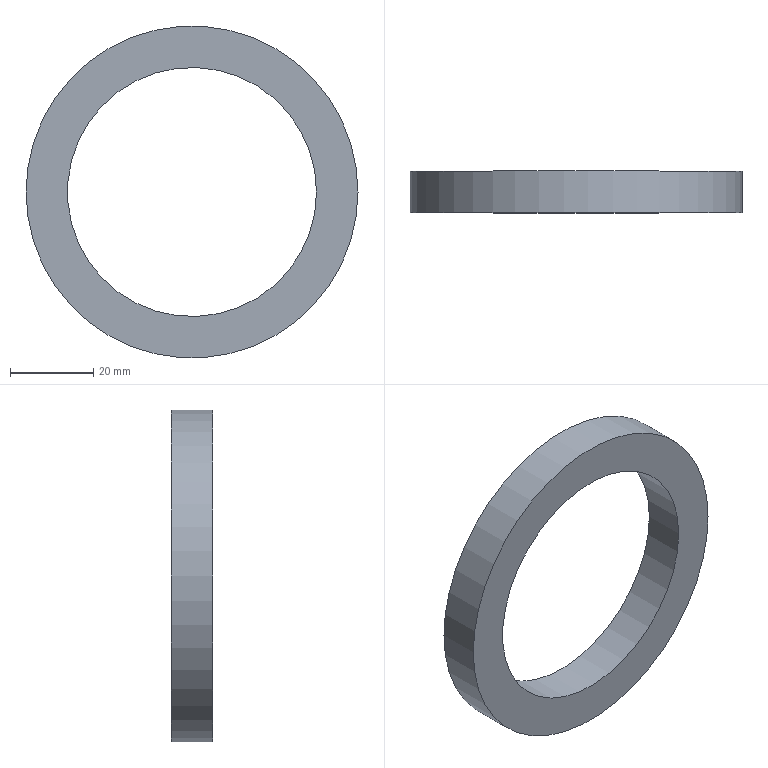Component | NX | OIL_SEAL_80X60X10 | 1 solid | 4 faces | box 80 x 10 x 80 mm | volume 21991 mm3 | cylinder 2 | plane 2 | commonest cylinder face diameters 80 x1 60 x1
STEP:
#1=CARTESIAN_POINT('',(0.,0.,0.));
#2=DIRECTION('',(0.,0.,1.));
#3=DIRECTION('',(1.,0.,0.));
#4=AXIS2_PLACEMENT_3D('',#1,#2,#3);
#5=CARTESIAN_POINT('',(45.,-94.6,-249.5));
#6=VERTEX_POINT('',#5);
#7=CARTESIAN_POINT('',(5.,-94.6,-249.5));
#8=DIRECTION('',(0.,-1.,0.));
#9=DIRECTION('',(1.,0.,0.));
#10=AXIS2_PLACEMENT_3D('',#7,#8,#9);
#11=CIRCLE('',#10,40.);
#12=CARTESIAN_POINT('',(5.,-94.6,-249.5));
#13=DIRECTION('',(0.,1.,0.));
#14=DIRECTION('',(-1.,0.,0.));
#15=AXIS2_PLACEMENT_3D('',#12,#13,#14);
#16=CYLINDRICAL_SURFACE('',#15,40.);
#17=CARTESIAN_POINT('',(9.425,0.));
#18=DIRECTION('',(-1.,0.));
#19=VECTOR('',#18,1.);
#20=LINE('',#17,#19);
#21=(GEOMETRIC_REPRESENTATION_CONTEXT(2)PARAMETRIC_REPRESENTATION_CONTEXT()REPRESENTATION_CONTEXT('',''));
#22=DEFINITIONAL_REPRESENTATION('',(#20),#21);
#23=PCURVE('',#16,#22);
#24=CARTESIAN_POINT('',(5.,-94.6,-249.5));
#25=DIRECTION('',(0.,-1.,0.));
#26=DIRECTION('',(1.,0.,0.));
#27=AXIS2_PLACEMENT_3D('',#24,#25,#26);
#28=PLANE('',#27);
#29=CARTESIAN_POINT('',(0.,0.));
#30=DIRECTION('',(1.,0.));
#31=AXIS2_PLACEMENT_2D('',#29,#30);
#32=CIRCLE('',#31,40.);
#33=(GEOMETRIC_REPRESENTATION_CONTEXT(2)PARAMETRIC_REPRESENTATION_CONTEXT()REPRESENTATION_CONTEXT('',''));
#34=DEFINITIONAL_REPRESENTATION('',(#32),#33);
#35=PCURVE('',#28,#34);
#36=SURFACE_CURVE('',#11,(#23,#35),.PCURVE_S1.);
#37=EDGE_CURVE('',#6,#6,#36,.T.);
#38=ORIENTED_EDGE('',*,*,#37,.F.);
#39=CARTESIAN_POINT('',(45.,-84.6,-249.5));
#40=VERTEX_POINT('',#39);
#41=CARTESIAN_POINT('',(45.,-94.6,-249.5));
#42=CARTESIAN_POINT('',(45.,-84.6,-249.5));
#43=B_SPLINE_CURVE_WITH_KNOTS('',1,(#41,#42),.UNSPECIFIED.,.F.,.F.,(2,2),(0.,10.),.PIECEWISE_BEZIER_KNOTS.);
#44=CARTESIAN_POINT('',(9.425,0.));
#45=DIRECTION('',(0.,1.));
#46=VECTOR('',#45,1.);
#47=LINE('',#44,#46);
#48=(GEOMETRIC_REPRESENTATION_CONTEXT(2)PARAMETRIC_REPRESENTATION_CONTEXT()REPRESENTATION_CONTEXT('',''));
#49=DEFINITIONAL_REPRESENTATION('',(#47),#48);
#50=PCURVE('',#16,#49);
#51=CARTESIAN_POINT('',(3.142,0.));
#52=DIRECTION('',(0.,1.));
#53=VECTOR('',#52,1.);
#54=LINE('',#51,#53);
#55=(GEOMETRIC_REPRESENTATION_CONTEXT(2)PARAMETRIC_REPRESENTATION_CONTEXT()REPRESENTATION_CONTEXT('',''));
#56=DEFINITIONAL_REPRESENTATION('',(#54),#55);
#57=PCURVE('',#16,#56);
#58=SEAM_CURVE('',#43,(#50,#57),.PCURVE_S1.);
#59=EDGE_CURVE('',#6,#40,#58,.T.);
#60=ORIENTED_EDGE('',*,*,#59,.T.);
#61=CARTESIAN_POINT('',(5.,-84.6,-249.5));
#62=DIRECTION('',(0.,-1.,0.));
#63=DIRECTION('',(1.,0.,0.));
#64=AXIS2_PLACEMENT_3D('',#61,#62,#63);
#65=CIRCLE('',#64,40.);
#66=CARTESIAN_POINT('',(9.425,10.));
#67=DIRECTION('',(-1.,0.));
#68=VECTOR('',#67,1.);
#69=LINE('',#66,#68);
#70=(GEOMETRIC_REPRESENTATION_CONTEXT(2)PARAMETRIC_REPRESENTATION_CONTEXT()REPRESENTATION_CONTEXT('',''));
#71=DEFINITIONAL_REPRESENTATION('',(#69),#70);
#72=PCURVE('',#16,#71);
#73=CARTESIAN_POINT('',(5.,-84.6,-249.5));
#74=DIRECTION('',(0.,-1.,0.));
#75=DIRECTION('',(1.,0.,0.));
#76=AXIS2_PLACEMENT_3D('',#73,#74,#75);
#77=PLANE('',#76);
#78=CARTESIAN_POINT('',(0.,0.));
#79=DIRECTION('',(1.,0.));
#80=AXIS2_PLACEMENT_2D('',#78,#79);
#81=CIRCLE('',#80,40.);
#82=(GEOMETRIC_REPRESENTATION_CONTEXT(2)PARAMETRIC_REPRESENTATION_CONTEXT()REPRESENTATION_CONTEXT('',''));
#83=DEFINITIONAL_REPRESENTATION('',(#81),#82);
#84=PCURVE('',#77,#83);
#85=SURFACE_CURVE('',#65,(#72,#84),.PCURVE_S1.);
#86=EDGE_CURVE('',#40,#40,#85,.T.);
#87=ORIENTED_EDGE('',*,*,#86,.T.);
#88=ORIENTED_EDGE('',*,*,#59,.F.);
#89=EDGE_LOOP('',(#38,#60,#87,#88));
#90=FACE_BOUND('',#89,.T.);
#91=ADVANCED_FACE('',(#90),#16,.T.);
#92=CARTESIAN_POINT('',(35.,-94.6,-249.5));
#93=VERTEX_POINT('',#92);
#94=CARTESIAN_POINT('',(5.,-94.6,-249.5));
#95=DIRECTION('',(0.,-1.,0.));
#96=DIRECTION('',(1.,0.,0.));
#97=AXIS2_PLACEMENT_3D('',#94,#95,#96);
#98=CIRCLE('',#97,30.);
#99=CARTESIAN_POINT('',(5.,-94.6,-249.5));
#100=DIRECTION('',(0.,1.,0.));
#101=DIRECTION('',(-1.,0.,0.));
#102=AXIS2_PLACEMENT_3D('',#99,#100,#101);
#103=CYLINDRICAL_SURFACE('',#102,30.);
#104=CARTESIAN_POINT('',(9.425,0.));
#105=DIRECTION('',(-1.,0.));
#106=VECTOR('',#105,1.);
#107=LINE('',#104,#106);
#108=(GEOMETRIC_REPRESENTATION_CONTEXT(2)PARAMETRIC_REPRESENTATION_CONTEXT()REPRESENTATION_CONTEXT('',''));
#109=DEFINITIONAL_REPRESENTATION('',(#107),#108);
#110=PCURVE('',#103,#109);
#111=CARTESIAN_POINT('',(0.,0.));
#112=DIRECTION('',(1.,0.));
#113=AXIS2_PLACEMENT_2D('',#111,#112);
#114=CIRCLE('',#113,30.);
#115=(GEOMETRIC_REPRESENTATION_CONTEXT(2)PARAMETRIC_REPRESENTATION_CONTEXT()REPRESENTATION_CONTEXT('',''));
#116=DEFINITIONAL_REPRESENTATION('',(#114),#115);
#117=PCURVE('',#28,#116);
#118=SURFACE_CURVE('',#98,(#110,#117),.PCURVE_S1.);
#119=EDGE_CURVE('',#93,#93,#118,.T.);
#120=ORIENTED_EDGE('',*,*,#119,.F.);
#121=CARTESIAN_POINT('',(35.,-84.6,-249.5));
#122=VERTEX_POINT('',#121);
#123=CARTESIAN_POINT('',(35.,-94.6,-249.5));
#124=CARTESIAN_POINT('',(35.,-84.6,-249.5));
#125=B_SPLINE_CURVE_WITH_KNOTS('',1,(#123,#124),.UNSPECIFIED.,.F.,.F.,(2,2),(0.,10.),.PIECEWISE_BEZIER_KNOTS.);
#126=CARTESIAN_POINT('',(9.425,0.));
#127=DIRECTION('',(0.,1.));
#128=VECTOR('',#127,1.);
#129=LINE('',#126,#128);
#130=(GEOMETRIC_REPRESENTATION_CONTEXT(2)PARAMETRIC_REPRESENTATION_CONTEXT()REPRESENTATION_CONTEXT('',''));
#131=DEFINITIONAL_REPRESENTATION('',(#129),#130);
#132=PCURVE('',#103,#131);
#133=CARTESIAN_POINT('',(3.142,0.));
#134=DIRECTION('',(0.,1.));
#135=VECTOR('',#134,1.);
#136=LINE('',#133,#135);
#137=(GEOMETRIC_REPRESENTATION_CONTEXT(2)PARAMETRIC_REPRESENTATION_CONTEXT()REPRESENTATION_CONTEXT('',''));
#138=DEFINITIONAL_REPRESENTATION('',(#136),#137);
#139=PCURVE('',#103,#138);
#140=SEAM_CURVE('',#125,(#132,#139),.PCURVE_S1.);
#141=EDGE_CURVE('',#93,#122,#140,.T.);
#142=ORIENTED_EDGE('',*,*,#141,.T.);
#143=CARTESIAN_POINT('',(5.,-84.6,-249.5));
#144=DIRECTION('',(0.,-1.,0.));
#145=DIRECTION('',(1.,0.,0.));
#146=AXIS2_PLACEMENT_3D('',#143,#144,#145);
#147=CIRCLE('',#146,30.);
#148=CARTESIAN_POINT('',(9.425,10.));
#149=DIRECTION('',(-1.,0.));
#150=VECTOR('',#149,1.);
#151=LINE('',#148,#150);
#152=(GEOMETRIC_REPRESENTATION_CONTEXT(2)PARAMETRIC_REPRESENTATION_CONTEXT()REPRESENTATION_CONTEXT('',''));
#153=DEFINITIONAL_REPRESENTATION('',(#151),#152);
#154=PCURVE('',#103,#153);
#155=CARTESIAN_POINT('',(0.,0.));
#156=DIRECTION('',(1.,0.));
#157=AXIS2_PLACEMENT_2D('',#155,#156);
#158=CIRCLE('',#157,30.);
#159=(GEOMETRIC_REPRESENTATION_CONTEXT(2)PARAMETRIC_REPRESENTATION_CONTEXT()REPRESENTATION_CONTEXT('',''));
#160=DEFINITIONAL_REPRESENTATION('',(#158),#159);
#161=PCURVE('',#77,#160);
#162=SURFACE_CURVE('',#147,(#154,#161),.PCURVE_S1.);
#163=EDGE_CURVE('',#122,#122,#162,.T.);
#164=ORIENTED_EDGE('',*,*,#163,.T.);
#165=ORIENTED_EDGE('',*,*,#141,.F.);
#166=EDGE_LOOP('',(#120,#142,#164,#165));
#167=FACE_BOUND('',#166,.F.);
#168=ADVANCED_FACE('',(#167),#103,.F.);
#169=ORIENTED_EDGE('',*,*,#37,.T.);
#170=EDGE_LOOP('',(#169));
#171=FACE_BOUND('',#170,.T.);
#172=ORIENTED_EDGE('',*,*,#119,.F.);
#173=EDGE_LOOP('',(#172));
#174=FACE_BOUND('',#173,.T.);
#175=ADVANCED_FACE('',(#171,#174),#28,.T.);
#176=ORIENTED_EDGE('',*,*,#86,.F.);
#177=EDGE_LOOP('',(#176));
#178=FACE_BOUND('',#177,.T.);
#179=ORIENTED_EDGE('',*,*,#163,.T.);
#180=EDGE_LOOP('',(#179));
#181=FACE_BOUND('',#180,.T.);
#182=ADVANCED_FACE('',(#178,#181),#77,.F.);
#183=CLOSED_SHELL('',(#91,#168,#175,#182));
#184=MANIFOLD_SOLID_BREP('',#183);
#185=(LENGTH_UNIT()NAMED_UNIT(*)SI_UNIT(.MILLI.,.METRE.));
#186=UNCERTAINTY_MEASURE_WITH_UNIT(LENGTH_MEASURE(0.00001),#185,'','');
#187=(NAMED_UNIT(*)PLANE_ANGLE_UNIT()SI_UNIT($,.RADIAN.));
#188=(NAMED_UNIT(*)SI_UNIT($,.STERADIAN.)SOLID_ANGLE_UNIT());
#189=(GEOMETRIC_REPRESENTATION_CONTEXT(3)GLOBAL_UNCERTAINTY_ASSIGNED_CONTEXT((#186))GLOBAL_UNIT_ASSIGNED_CONTEXT((#185,#187,#188))REPRESENTATION_CONTEXT('',''));
#190=ADVANCED_BREP_SHAPE_REPRESENTATION('',(#4,#184),#189);